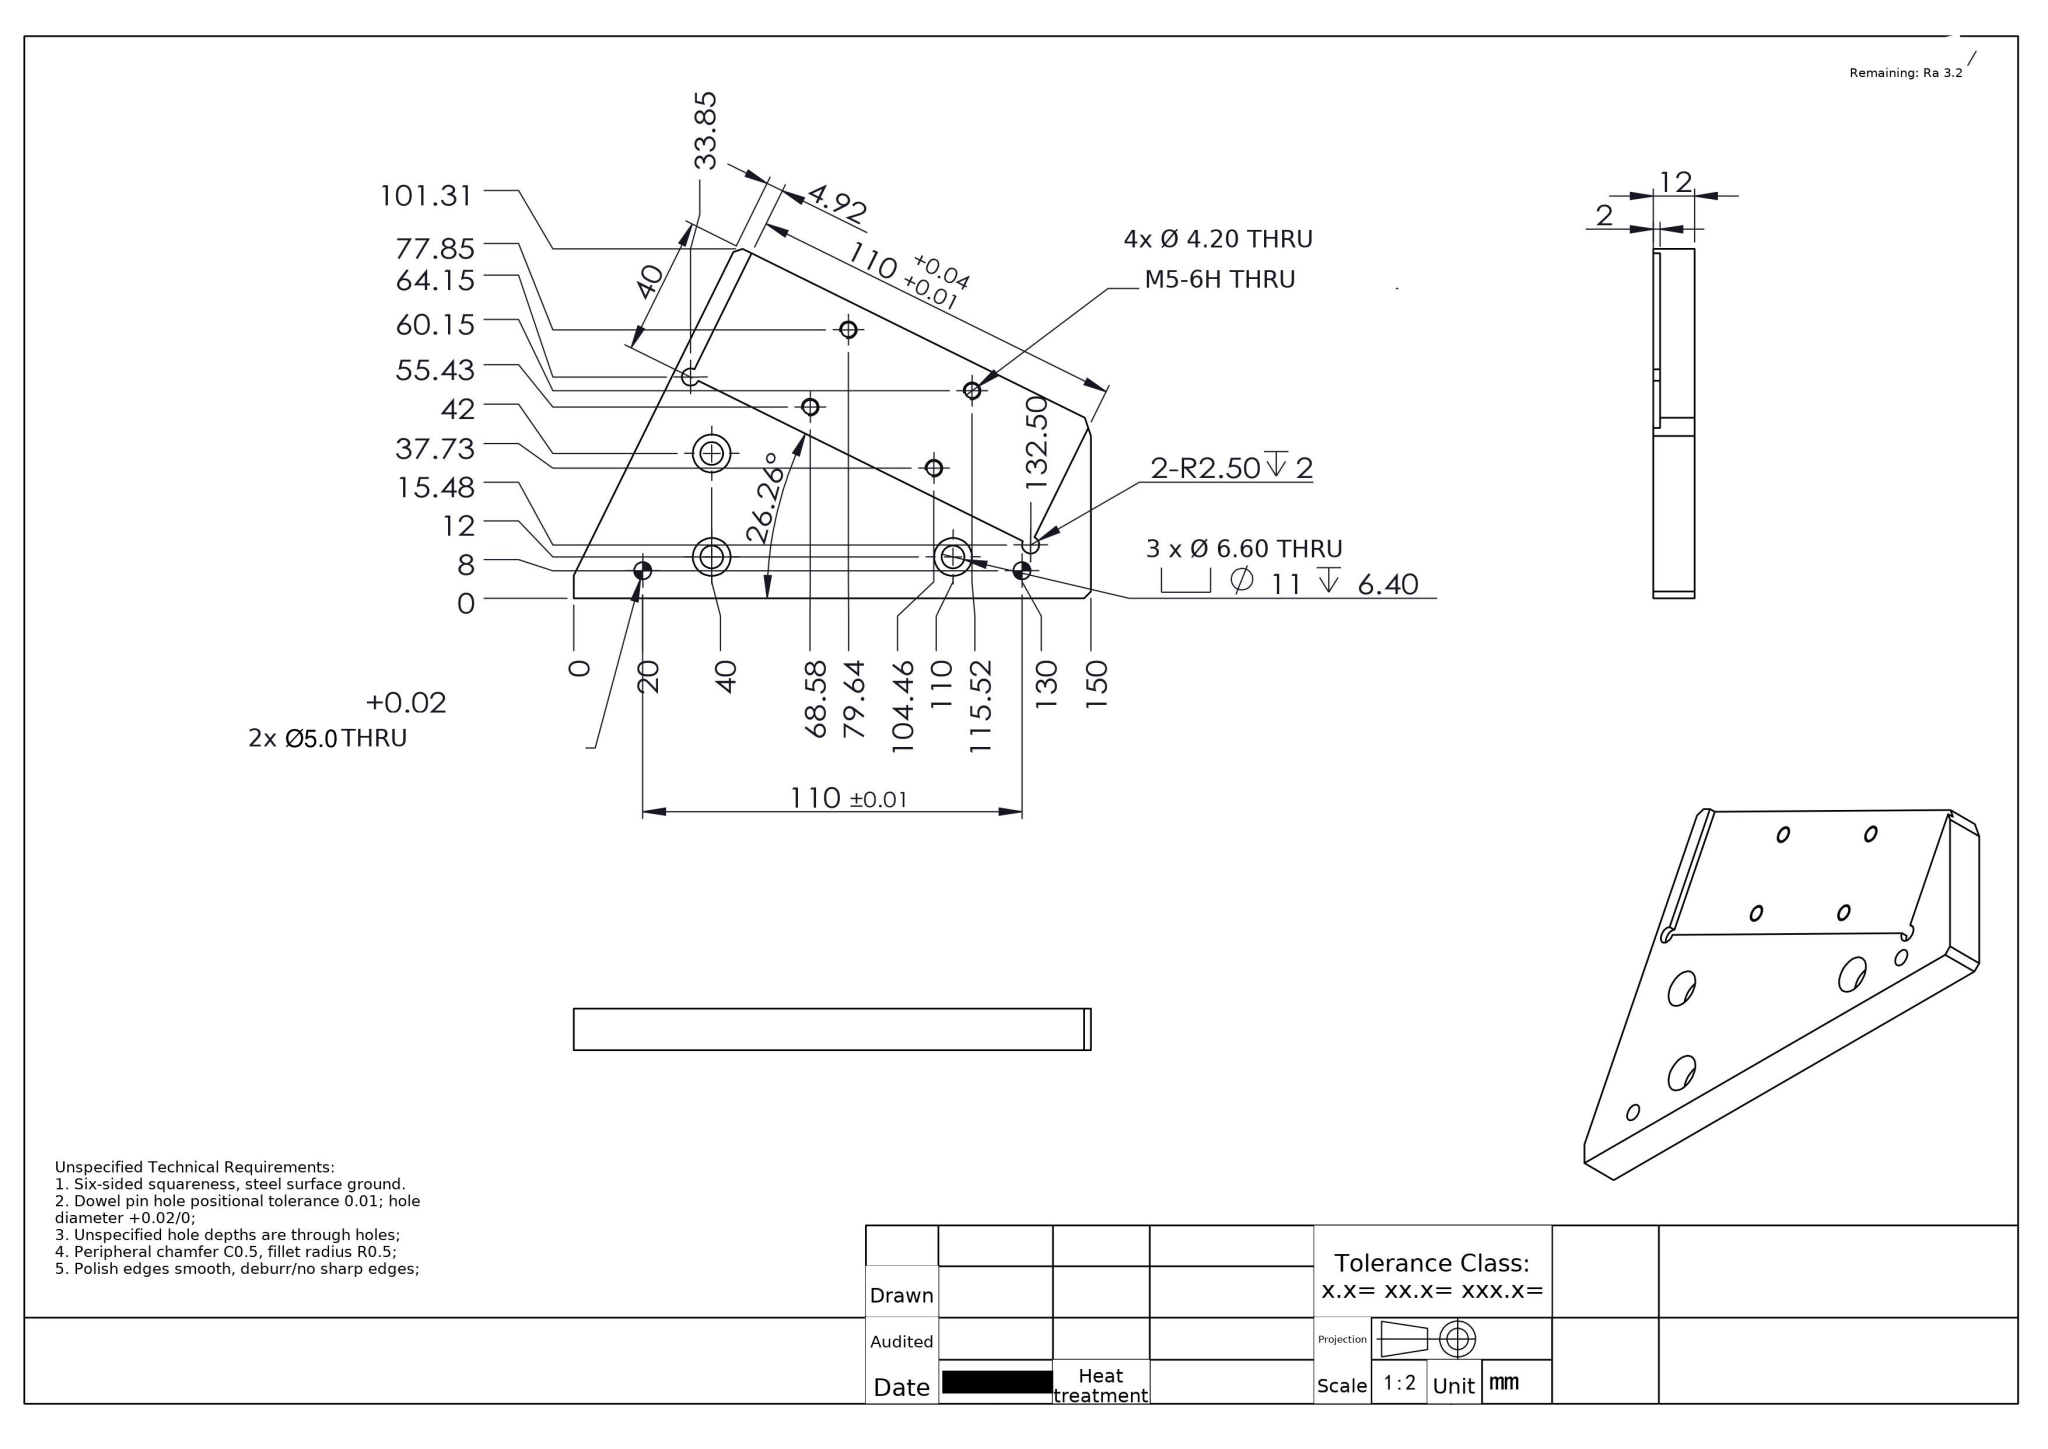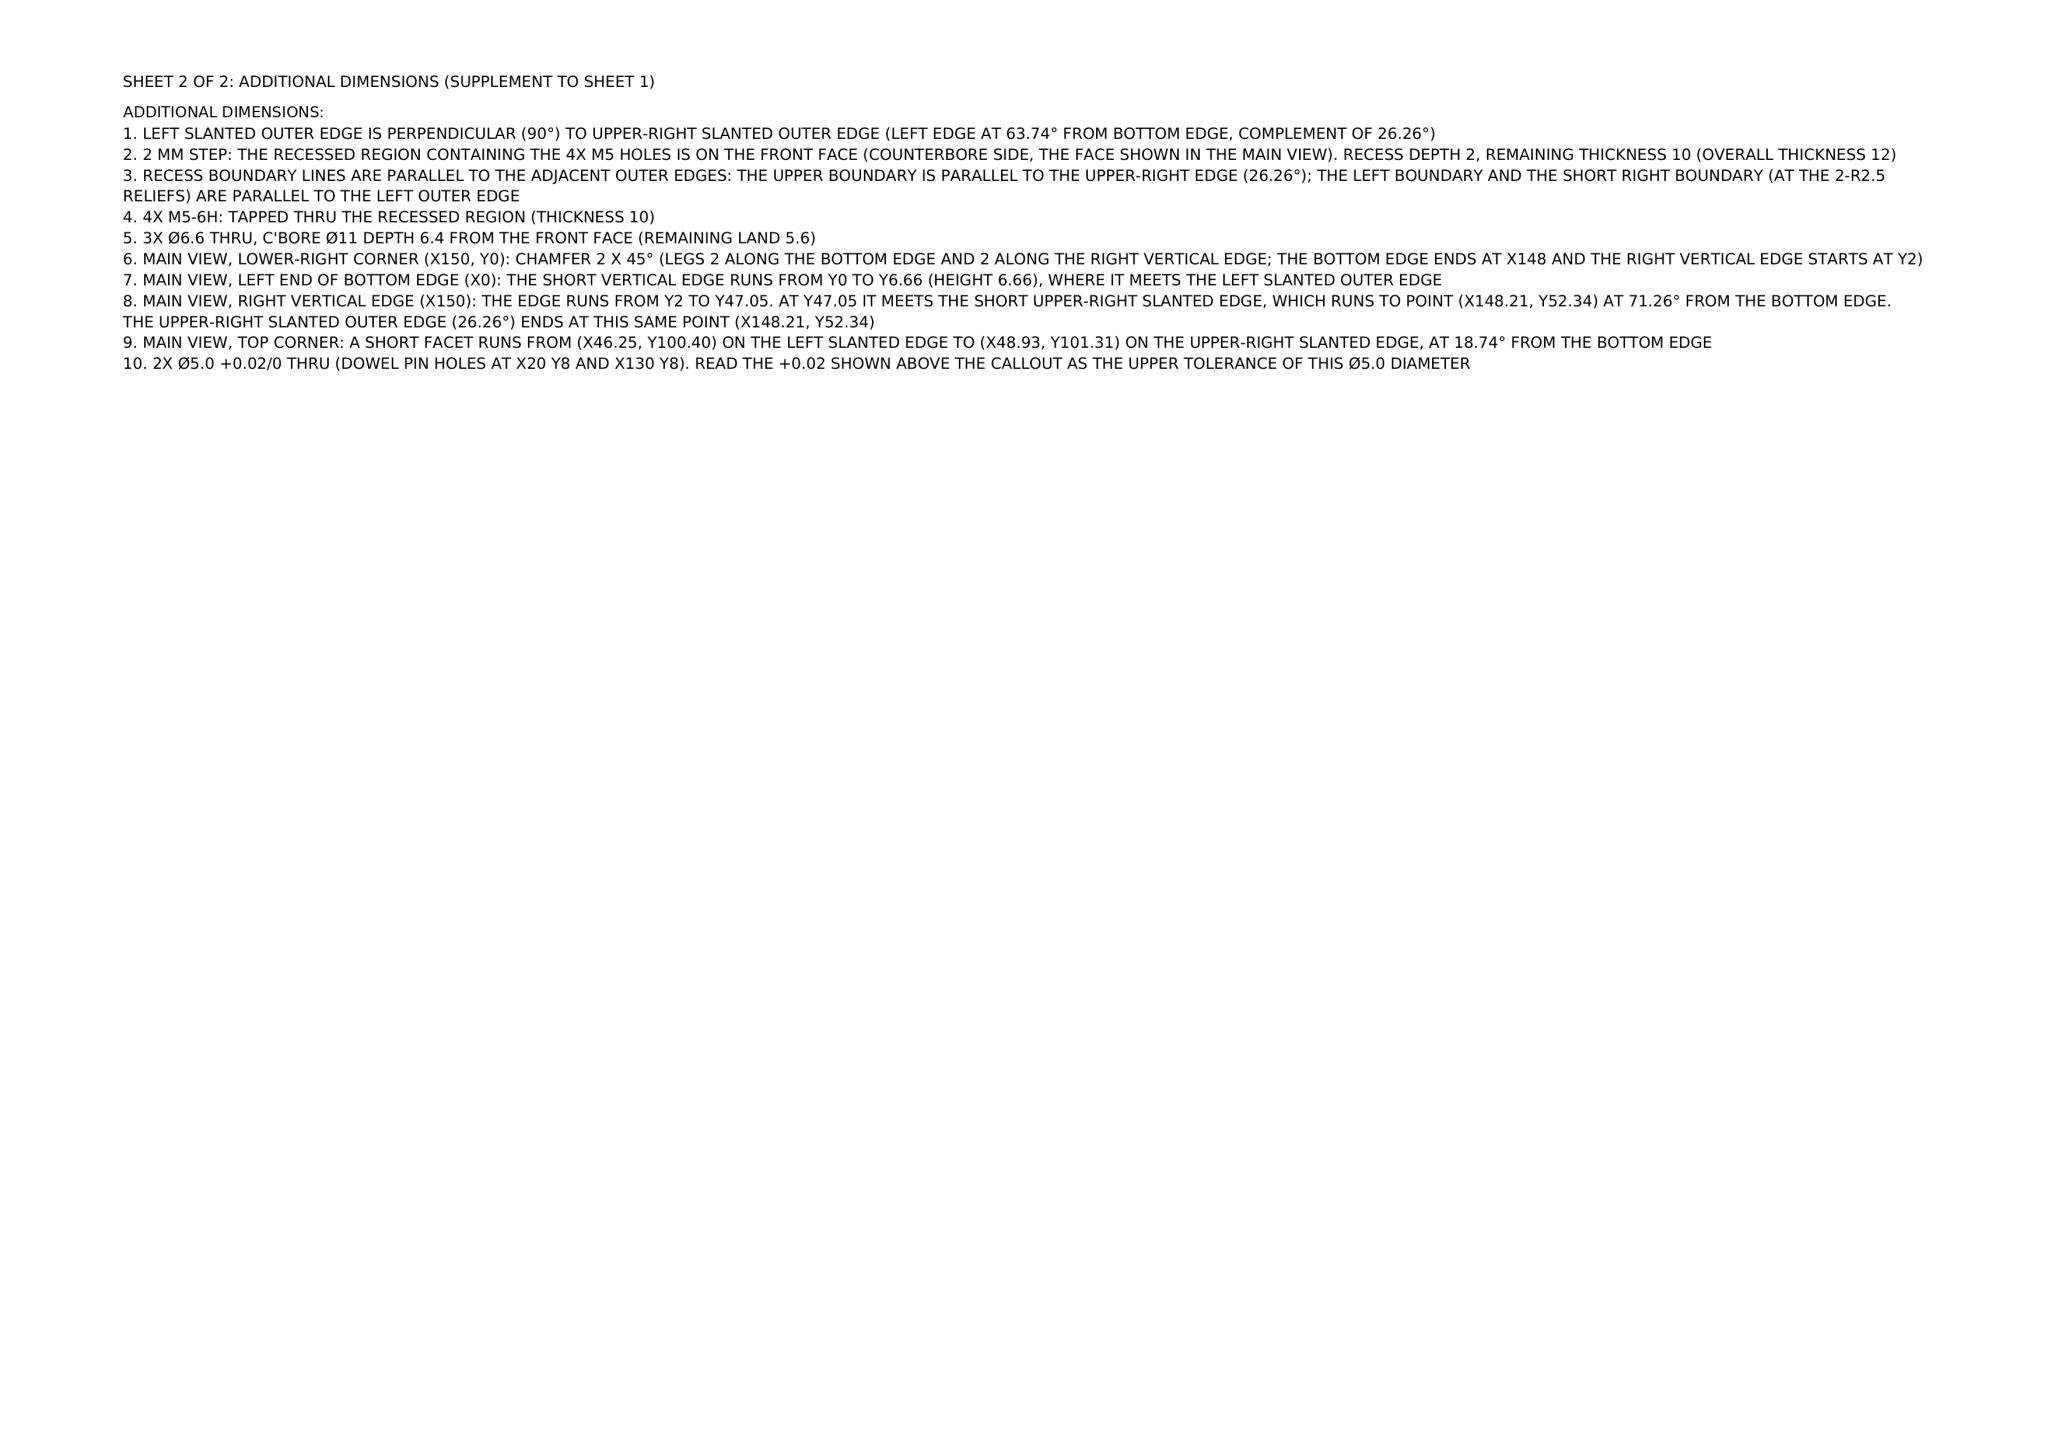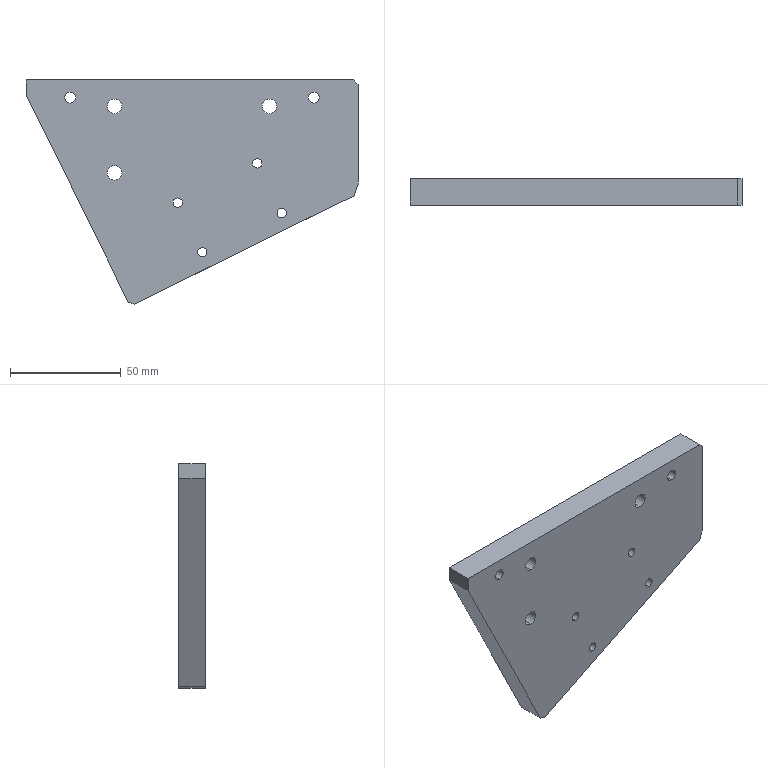Part | NX | mm | 1 solid | 46 faces | box 150 x 12 x 101.31 mm | volume 113235 mm3 | cylinder 29 | plane 17 | commonest cylinder face diameters 5 x9 4.2 x8 11 x6 6.6 x6